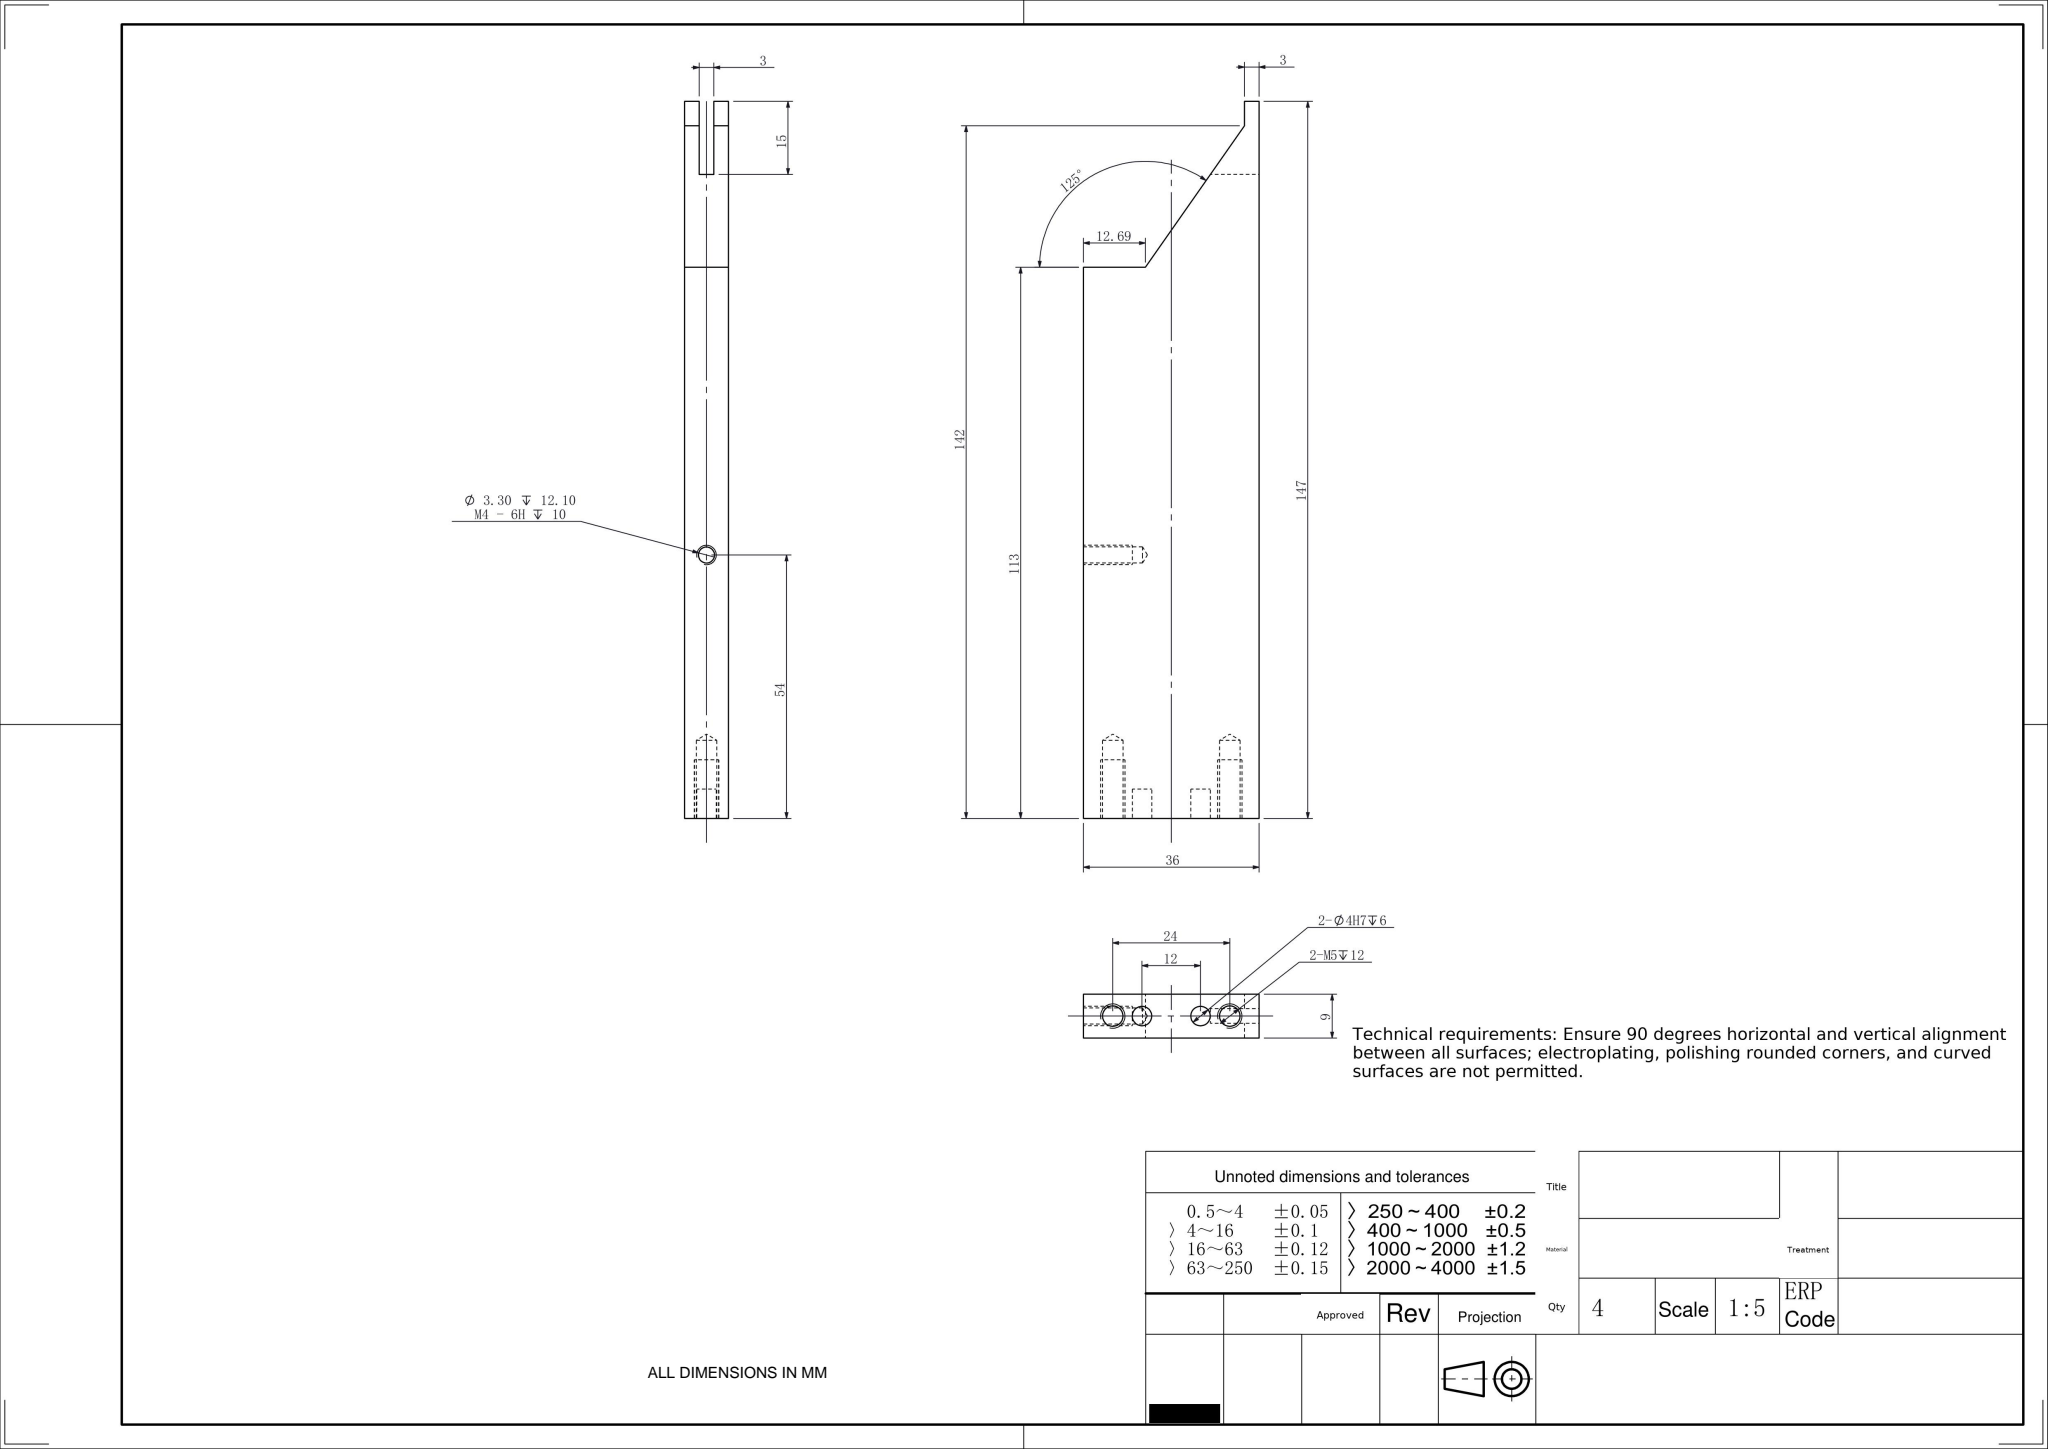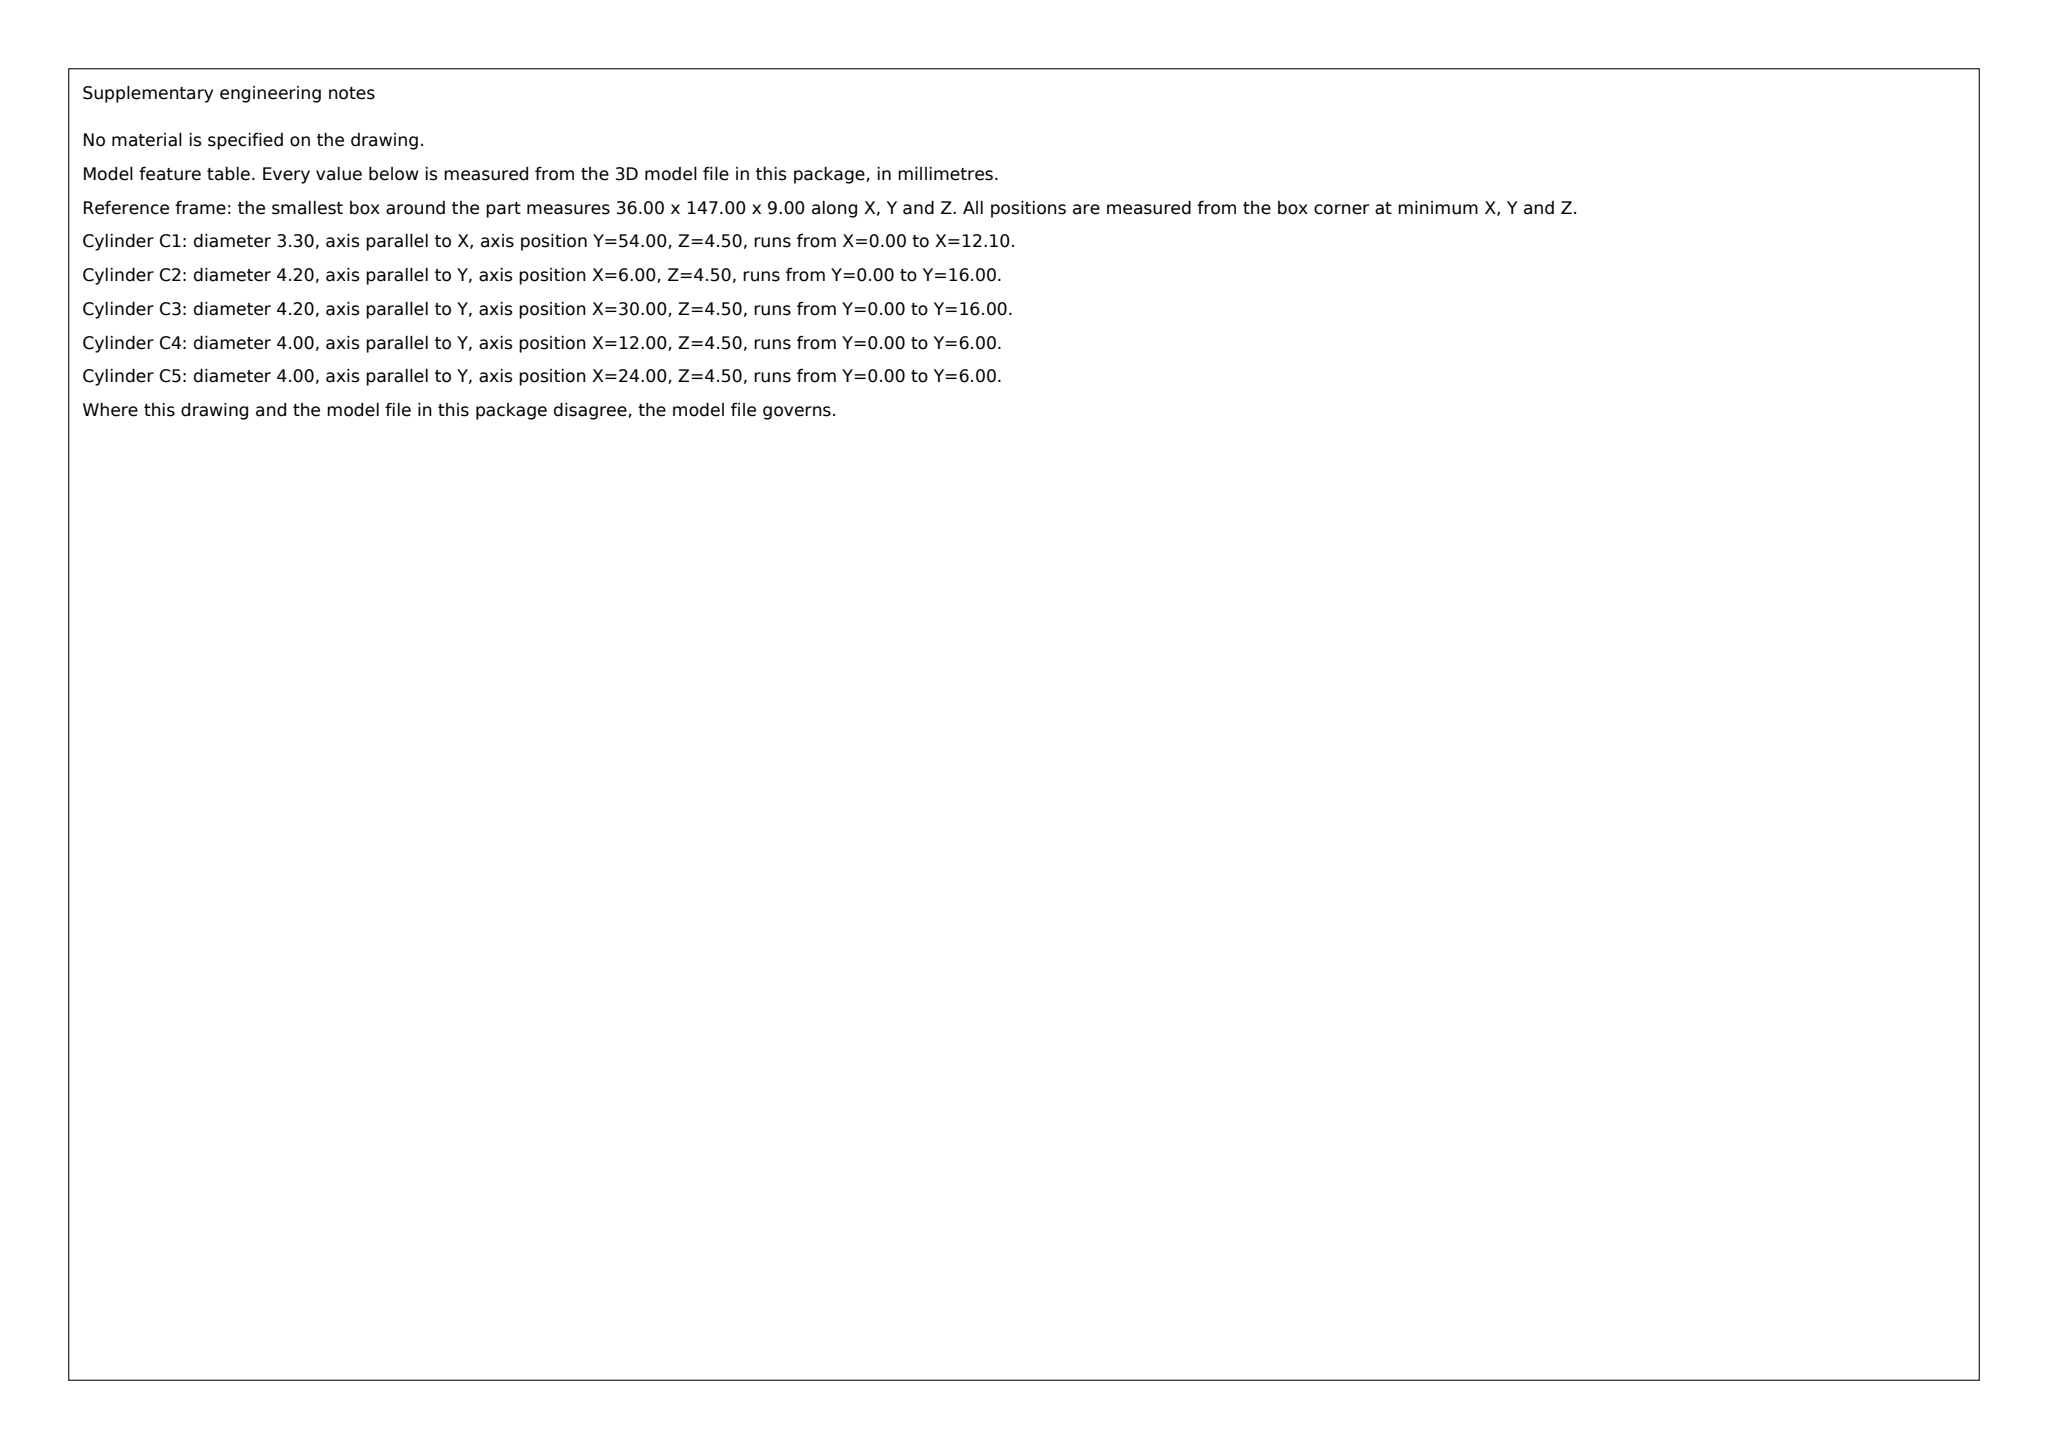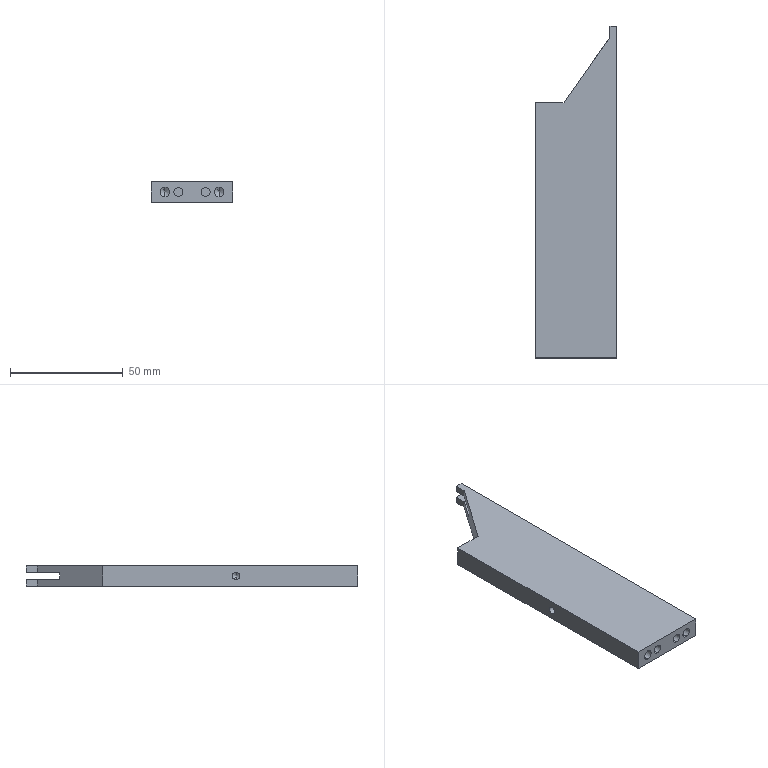Part | SolidWorks | mm | 1 solid | 32 faces | box 36 x 147 x 9 mm | volume 39228 mm3 | plane 16 | cylinder 10 | cone 6 | commonest cylinder face diameters 4 x4 4.2 x4 3.3 x2
build123d program:
from build123d import *

# Parameters (mm, degrees)
SKETCH1_W             = 36
SKETCH1_H             = 147
BOSS_EXTRUDE1_DEPTH   = 9
M5_TAPPED_HOLE1_D     = 4.2
M5_TAPPED_HOLE1_DEPTH = 16
M5_TAPPED_HOLE1_TIP   = 1.262
SKETCH3_R             = 2
CUT_EXTRUDE1_DEPTH    = 6
M4_TAPPED_HOLE1_D     = 3.3
M4_TAPPED_HOLE1_DEPTH = 12.1
M4_TAPPED_HOLE1_TIP   = 0.9914
CUT_EXTRUDE2_DEPTH    = 149.371
SKETCH8_W             = 3
SKETCH8_H             = 15
CUT_EXTRUDE3_DEPTH    = 152.611


with BuildPart() as part:
    # Sketch1 → Boss-Extrude1 (new body)
    with BuildSketch(Plane.XY):
        with Locations((0, 73.5)):
            Rectangle(SKETCH1_W, SKETCH1_H)
    extrude(amount=BOSS_EXTRUDE1_DEPTH)

    # M5 Tapped Hole1
    with Locations(Plane(origin=(-12, 0, 4.5), x_dir=(0, 0, -1), z_dir=(0, -1, 0))):
        with Locations((0, 0), (0, 24)):
            Hole(M5_TAPPED_HOLE1_D / 2, depth=M5_TAPPED_HOLE1_DEPTH)
            with Locations((0, 0, -(M5_TAPPED_HOLE1_DEPTH + M5_TAPPED_HOLE1_TIP / 2))):  # 118° drill point
                Cone(0, M5_TAPPED_HOLE1_D / 2, M5_TAPPED_HOLE1_TIP, mode=Mode.SUBTRACT)

    # Sketch3 → Cut-Extrude1 (cut)
    with BuildSketch(Plane.XZ):
        with Locations(Location((-6, 4.5, 0), (0, 0, 270))):
            Circle(SKETCH3_R)
        with Locations(Location((6, 4.5, 0), (0, 0, 270))):
            Circle(SKETCH3_R)
    extrude(amount=-CUT_EXTRUDE1_DEPTH, mode=Mode.SUBTRACT)

    # M4 Tapped Hole1
    with Locations(Plane(origin=(-18, 54, 4.5), x_dir=(0, 0, -1), z_dir=(-1, 0, 0))):
        with Locations((0, 0)):
            Hole(M4_TAPPED_HOLE1_D / 2, depth=M4_TAPPED_HOLE1_DEPTH)
            with Locations((0, 0, -(M4_TAPPED_HOLE1_DEPTH + M4_TAPPED_HOLE1_TIP / 2))):  # 118° drill point
                Cone(0, M4_TAPPED_HOLE1_D / 2, M4_TAPPED_HOLE1_TIP, mode=Mode.SUBTRACT)

    # Sketch6 → Cut-Extrude2 (cut, through all)
    with BuildSketch(Plane.XY.offset(9)):
        Polygon((15, 147), (-44.648, 147), (-44.648, 113), (-5.306, 113), (15, 142), align=None)
    extrude(amount=-CUT_EXTRUDE2_DEPTH, mode=Mode.SUBTRACT)

    # Sketch8 → Cut-Extrude3 (cut, through all)
    with BuildSketch(Plane(origin=(18, 0, 0), x_dir=(0, 0, -1), z_dir=(1, 0, 0))):
        with Locations((-4.5, 139.5)):
            Rectangle(SKETCH8_W, SKETCH8_H)
    extrude(amount=-CUT_EXTRUDE3_DEPTH, mode=Mode.SUBTRACT)


solid = part.part
STEP:
#1=CARTESIAN_POINT('',(-5.9,54.,2.85));
#2=VERTEX_POINT('',#1);
#3=CARTESIAN_POINT('',(-5.9,54.,6.15));
#4=VERTEX_POINT('',#3);
#5=CARTESIAN_POINT('',(-5.9,54.,4.5));
#6=DIRECTION('',(-1.,0.,0.));
#7=DIRECTION('',(0.,0.,1.));
#8=AXIS2_PLACEMENT_3D('',#5,#6,#7);
#9=CIRCLE('',#8,1.65);
#10=EDGE_CURVE('',#2,#4,#9,.T.);
#11=ORIENTED_EDGE('',*,*,#10,.F.);
#12=CARTESIAN_POINT('',(-18.,54.,2.85));
#13=VERTEX_POINT('',#12);
#14=CARTESIAN_POINT('',(-18.,54.,2.85));
#15=DIRECTION('',(-1.,0.,0.));
#16=VECTOR('',#15,1000.);
#17=LINE('',#14,#16);
#18=EDGE_CURVE('',#2,#13,#17,.T.);
#19=ORIENTED_EDGE('',*,*,#18,.T.);
#20=CARTESIAN_POINT('',(-18.,54.,6.15));
#21=VERTEX_POINT('',#20);
#22=CARTESIAN_POINT('',(-18.,54.,4.5));
#23=DIRECTION('',(-1.,0.,0.));
#24=DIRECTION('',(0.,0.,1.));
#25=AXIS2_PLACEMENT_3D('',#22,#23,#24);
#26=CIRCLE('',#25,1.65);
#27=EDGE_CURVE('',#13,#21,#26,.T.);
#28=ORIENTED_EDGE('',*,*,#27,.T.);
#29=CARTESIAN_POINT('',(-18.,54.,6.15));
#30=DIRECTION('',(-1.,0.,0.));
#31=VECTOR('',#30,1000.);
#32=LINE('',#29,#31);
#33=EDGE_CURVE('',#4,#21,#32,.T.);
#34=ORIENTED_EDGE('',*,*,#33,.F.);
#35=EDGE_LOOP('',(#11,#19,#28,#34));
#36=FACE_OUTER_BOUND('',#35,.T.);
#37=CARTESIAN_POINT('',(-18.,54.,4.5));
#38=DIRECTION('',(-1.,0.,0.));
#39=DIRECTION('',(0.,0.,1.));
#40=AXIS2_PLACEMENT_3D('',#37,#38,#39);
#41=CYLINDRICAL_SURFACE('',#40,1.65);
#42=ADVANCED_FACE('',(#36),#41,.F.);
#43=CARTESIAN_POINT('',(-4.909,54.,4.5));
#44=VERTEX_POINT('',#43);
#45=CARTESIAN_POINT('',(-5.9,54.,6.15));
#46=DIRECTION('',(-0.515,0.,0.8572));
#47=VECTOR('',#46,1000.);
#48=LINE('',#45,#47);
#49=EDGE_CURVE('',#44,#4,#48,.T.);
#50=ORIENTED_EDGE('',*,*,#49,.F.);
#51=CARTESIAN_POINT('',(-5.9,54.,2.85));
#52=DIRECTION('',(-0.515,0.,-0.8572));
#53=VECTOR('',#52,1000.);
#54=LINE('',#51,#53);
#55=EDGE_CURVE('',#44,#2,#54,.T.);
#56=ORIENTED_EDGE('',*,*,#55,.T.);
#57=ORIENTED_EDGE('',*,*,#10,.T.);
#58=EDGE_LOOP('',(#50,#56,#57));
#59=FACE_OUTER_BOUND('',#58,.T.);
#60=CARTESIAN_POINT('',(-5.9,54.,4.5));
#61=DIRECTION('',(-1.,0.,0.));
#62=DIRECTION('',(0.,0.,1.));
#63=AXIS2_PLACEMENT_3D('',#60,#61,#62);
#64=CONICAL_SURFACE('',#63,1.65,1.03);
#65=ADVANCED_FACE('',(#59),#64,.F.);
#66=CARTESIAN_POINT('',(6.,6.,6.5));
#67=VERTEX_POINT('',#66);
#68=CARTESIAN_POINT('',(6.,6.,2.5));
#69=VERTEX_POINT('',#68);
#70=CARTESIAN_POINT('',(6.,6.,4.5));
#71=DIRECTION('',(0.,-1.,0.));
#72=DIRECTION('',(0.,0.,-1.));
#73=AXIS2_PLACEMENT_3D('',#70,#71,#72);
#74=CIRCLE('',#73,2.);
#75=EDGE_CURVE('',#67,#69,#74,.T.);
#76=ORIENTED_EDGE('',*,*,#75,.F.);
#77=CARTESIAN_POINT('',(6.,0.,6.5));
#78=VERTEX_POINT('',#77);
#79=CARTESIAN_POINT('',(6.,6.,6.5));
#80=DIRECTION('',(0.,-1.,0.));
#81=VECTOR('',#80,1000.);
#82=LINE('',#79,#81);
#83=EDGE_CURVE('',#67,#78,#82,.T.);
#84=ORIENTED_EDGE('',*,*,#83,.T.);
#85=CARTESIAN_POINT('',(6.,0.,2.5));
#86=VERTEX_POINT('',#85);
#87=CARTESIAN_POINT('',(6.,0.,4.5));
#88=DIRECTION('',(0.,-1.,0.));
#89=DIRECTION('',(0.,0.,-1.));
#90=AXIS2_PLACEMENT_3D('',#87,#88,#89);
#91=CIRCLE('',#90,2.);
#92=EDGE_CURVE('',#78,#86,#91,.T.);
#93=ORIENTED_EDGE('',*,*,#92,.T.);
#94=CARTESIAN_POINT('',(6.,6.,2.5));
#95=DIRECTION('',(0.,-1.,0.));
#96=VECTOR('',#95,1000.);
#97=LINE('',#94,#96);
#98=EDGE_CURVE('',#69,#86,#97,.T.);
#99=ORIENTED_EDGE('',*,*,#98,.F.);
#100=EDGE_LOOP('',(#76,#84,#93,#99));
#101=FACE_OUTER_BOUND('',#100,.T.);
#102=CARTESIAN_POINT('',(6.,6.,4.5));
#103=DIRECTION('',(0.,-1.,0.));
#104=DIRECTION('',(0.,0.,-1.));
#105=AXIS2_PLACEMENT_3D('',#102,#103,#104);
#106=CYLINDRICAL_SURFACE('',#105,2.);
#107=ADVANCED_FACE('',(#101),#106,.F.);
#108=CARTESIAN_POINT('',(-6.,6.,6.5));
#109=VERTEX_POINT('',#108);
#110=CARTESIAN_POINT('',(-6.,6.,2.5));
#111=VERTEX_POINT('',#110);
#112=CARTESIAN_POINT('',(-6.,6.,4.5));
#113=DIRECTION('',(0.,-1.,0.));
#114=DIRECTION('',(0.,0.,-1.));
#115=AXIS2_PLACEMENT_3D('',#112,#113,#114);
#116=CIRCLE('',#115,2.);
#117=EDGE_CURVE('',#109,#111,#116,.T.);
#118=ORIENTED_EDGE('',*,*,#117,.F.);
#119=CARTESIAN_POINT('',(-6.,0.,6.5));
#120=VERTEX_POINT('',#119);
#121=CARTESIAN_POINT('',(-6.,6.,6.5));
#122=DIRECTION('',(0.,-1.,0.));
#123=VECTOR('',#122,1000.);
#124=LINE('',#121,#123);
#125=EDGE_CURVE('',#109,#120,#124,.T.);
#126=ORIENTED_EDGE('',*,*,#125,.T.);
#127=CARTESIAN_POINT('',(-6.,0.,2.5));
#128=VERTEX_POINT('',#127);
#129=CARTESIAN_POINT('',(-6.,0.,4.5));
#130=DIRECTION('',(0.,-1.,0.));
#131=DIRECTION('',(0.,0.,-1.));
#132=AXIS2_PLACEMENT_3D('',#129,#130,#131);
#133=CIRCLE('',#132,2.);
#134=EDGE_CURVE('',#120,#128,#133,.T.);
#135=ORIENTED_EDGE('',*,*,#134,.T.);
#136=CARTESIAN_POINT('',(-6.,6.,2.5));
#137=DIRECTION('',(0.,-1.,0.));
#138=VECTOR('',#137,1000.);
#139=LINE('',#136,#138);
#140=EDGE_CURVE('',#111,#128,#139,.T.);
#141=ORIENTED_EDGE('',*,*,#140,.F.);
#142=EDGE_LOOP('',(#118,#126,#135,#141));
#143=FACE_OUTER_BOUND('',#142,.T.);
#144=CARTESIAN_POINT('',(-6.,6.,4.5));
#145=DIRECTION('',(0.,-1.,0.));
#146=DIRECTION('',(0.,0.,-1.));
#147=AXIS2_PLACEMENT_3D('',#144,#145,#146);
#148=CYLINDRICAL_SURFACE('',#147,2.);
#149=ADVANCED_FACE('',(#143),#148,.F.);
#150=CARTESIAN_POINT('',(-12.,16.,6.6));
#151=VERTEX_POINT('',#150);
#152=CARTESIAN_POINT('',(-12.,16.,2.4));
#153=VERTEX_POINT('',#152);
#154=CARTESIAN_POINT('',(-12.,16.,4.5));
#155=DIRECTION('',(0.,-1.,0.));
#156=DIRECTION('',(0.,0.,-1.));
#157=AXIS2_PLACEMENT_3D('',#154,#155,#156);
#158=CIRCLE('',#157,2.1);
#159=EDGE_CURVE('',#151,#153,#158,.T.);
#160=ORIENTED_EDGE('',*,*,#159,.F.);
#161=CARTESIAN_POINT('',(-12.,-0.,6.6));
#162=VERTEX_POINT('',#161);
#163=CARTESIAN_POINT('',(-12.,0.,6.6));
#164=DIRECTION('',(0.,-1.,0.));
#165=VECTOR('',#164,1000.);
#166=LINE('',#163,#165);
#167=EDGE_CURVE('',#151,#162,#166,.T.);
#168=ORIENTED_EDGE('',*,*,#167,.T.);
#169=CARTESIAN_POINT('',(-12.,-0.,2.4));
#170=VERTEX_POINT('',#169);
#171=CARTESIAN_POINT('',(-12.,-0.,4.5));
#172=DIRECTION('',(0.,-1.,0.));
#173=DIRECTION('',(0.,0.,-1.));
#174=AXIS2_PLACEMENT_3D('',#171,#172,#173);
#175=CIRCLE('',#174,2.1);
#176=EDGE_CURVE('',#162,#170,#175,.T.);
#177=ORIENTED_EDGE('',*,*,#176,.T.);
#178=CARTESIAN_POINT('',(-12.,0.,2.4));
#179=DIRECTION('',(0.,-1.,0.));
#180=VECTOR('',#179,1000.);
#181=LINE('',#178,#180);
#182=EDGE_CURVE('',#153,#170,#181,.T.);
#183=ORIENTED_EDGE('',*,*,#182,.F.);
#184=EDGE_LOOP('',(#160,#168,#177,#183));
#185=FACE_OUTER_BOUND('',#184,.T.);
#186=CARTESIAN_POINT('',(-12.,0.,4.5));
#187=DIRECTION('',(0.,-1.,0.));
#188=DIRECTION('',(0.,0.,-1.));
#189=AXIS2_PLACEMENT_3D('',#186,#187,#188);
#190=CYLINDRICAL_SURFACE('',#189,2.1);
#191=ADVANCED_FACE('',(#185),#190,.F.);
#192=CARTESIAN_POINT('',(-12.,17.262,4.5));
#193=VERTEX_POINT('',#192);
#194=CARTESIAN_POINT('',(-12.,16.,2.4));
#195=DIRECTION('',(0.,-0.515,-0.8572));
#196=VECTOR('',#195,1000.);
#197=LINE('',#194,#196);
#198=EDGE_CURVE('',#193,#153,#197,.T.);
#199=ORIENTED_EDGE('',*,*,#198,.F.);
#200=CARTESIAN_POINT('',(-12.,16.,6.6));
#201=DIRECTION('',(0.,-0.515,0.8572));
#202=VECTOR('',#201,1000.);
#203=LINE('',#200,#202);
#204=EDGE_CURVE('',#193,#151,#203,.T.);
#205=ORIENTED_EDGE('',*,*,#204,.T.);
#206=ORIENTED_EDGE('',*,*,#159,.T.);
#207=EDGE_LOOP('',(#199,#205,#206));
#208=FACE_OUTER_BOUND('',#207,.T.);
#209=CARTESIAN_POINT('',(-12.,16.,4.5));
#210=DIRECTION('',(0.,-1.,0.));
#211=DIRECTION('',(0.,0.,-1.));
#212=AXIS2_PLACEMENT_3D('',#209,#210,#211);
#213=CONICAL_SURFACE('',#212,2.1,1.03);
#214=ADVANCED_FACE('',(#208),#213,.F.);
#215=CARTESIAN_POINT('',(12.,16.,6.6));
#216=VERTEX_POINT('',#215);
#217=CARTESIAN_POINT('',(12.,16.,2.4));
#218=VERTEX_POINT('',#217);
#219=CARTESIAN_POINT('',(12.,16.,4.5));
#220=DIRECTION('',(0.,-1.,0.));
#221=DIRECTION('',(0.,0.,-1.));
#222=AXIS2_PLACEMENT_3D('',#219,#220,#221);
#223=CIRCLE('',#222,2.1);
#224=EDGE_CURVE('',#216,#218,#223,.T.);
#225=ORIENTED_EDGE('',*,*,#224,.F.);
#226=CARTESIAN_POINT('',(12.,-0.,6.6));
#227=VERTEX_POINT('',#226);
#228=CARTESIAN_POINT('',(12.,0.,6.6));
#229=DIRECTION('',(0.,-1.,0.));
#230=VECTOR('',#229,1000.);
#231=LINE('',#228,#230);
#232=EDGE_CURVE('',#216,#227,#231,.T.);
#233=ORIENTED_EDGE('',*,*,#232,.T.);
#234=CARTESIAN_POINT('',(12.,-0.,2.4));
#235=VERTEX_POINT('',#234);
#236=CARTESIAN_POINT('',(12.,-0.,4.5));
#237=DIRECTION('',(0.,-1.,0.));
#238=DIRECTION('',(0.,0.,-1.));
#239=AXIS2_PLACEMENT_3D('',#236,#237,#238);
#240=CIRCLE('',#239,2.1);
#241=EDGE_CURVE('',#227,#235,#240,.T.);
#242=ORIENTED_EDGE('',*,*,#241,.T.);
#243=CARTESIAN_POINT('',(12.,0.,2.4));
#244=DIRECTION('',(0.,-1.,0.));
#245=VECTOR('',#244,1000.);
#246=LINE('',#243,#245);
#247=EDGE_CURVE('',#218,#235,#246,.T.);
#248=ORIENTED_EDGE('',*,*,#247,.F.);
#249=EDGE_LOOP('',(#225,#233,#242,#248));
#250=FACE_OUTER_BOUND('',#249,.T.);
#251=CARTESIAN_POINT('',(12.,0.,4.5));
#252=DIRECTION('',(0.,-1.,0.));
#253=DIRECTION('',(0.,0.,-1.));
#254=AXIS2_PLACEMENT_3D('',#251,#252,#253);
#255=CYLINDRICAL_SURFACE('',#254,2.1);
#256=ADVANCED_FACE('',(#250),#255,.F.);
#257=CARTESIAN_POINT('',(12.,17.262,4.5));
#258=VERTEX_POINT('',#257);
#259=CARTESIAN_POINT('',(12.,16.,2.4));
#260=DIRECTION('',(0.,-0.515,-0.8572));
#261=VECTOR('',#260,1000.);
#262=LINE('',#259,#261);
#263=EDGE_CURVE('',#258,#218,#262,.T.);
#264=ORIENTED_EDGE('',*,*,#263,.F.);
#265=CARTESIAN_POINT('',(12.,16.,6.6));
#266=DIRECTION('',(0.,-0.515,0.8572));
#267=VECTOR('',#266,1000.);
#268=LINE('',#265,#267);
#269=EDGE_CURVE('',#258,#216,#268,.T.);
#270=ORIENTED_EDGE('',*,*,#269,.T.);
#271=ORIENTED_EDGE('',*,*,#224,.T.);
#272=EDGE_LOOP('',(#264,#270,#271));
#273=FACE_OUTER_BOUND('',#272,.T.);
#274=CARTESIAN_POINT('',(12.,16.,4.5));
#275=DIRECTION('',(0.,-1.,0.));
#276=DIRECTION('',(0.,0.,-1.));
#277=AXIS2_PLACEMENT_3D('',#274,#275,#276);
#278=CONICAL_SURFACE('',#277,2.1,1.03);
#279=ADVANCED_FACE('',(#273),#278,.F.);
#280=CARTESIAN_POINT('',(18.,147.,9.));
#281=VERTEX_POINT('',#280);
#282=CARTESIAN_POINT('',(18.,147.,6.));
#283=VERTEX_POINT('',#282);
#284=CARTESIAN_POINT('',(18.,147.,9.));
#285=DIRECTION('',(0.,0.,-1.));
#286=VECTOR('',#285,1000.);
#287=LINE('',#284,#286);
#288=EDGE_CURVE('',#281,#283,#287,.T.);
#289=ORIENTED_EDGE('',*,*,#288,.T.);
#290=CARTESIAN_POINT('',(15.,147.,6.));
#291=VERTEX_POINT('',#290);
#292=CARTESIAN_POINT('',(-18.,147.,6.));
#293=DIRECTION('',(1.,0.,0.));
#294=VECTOR('',#293,1000.);
#295=LINE('',#292,#294);
#296=EDGE_CURVE('',#291,#283,#295,.T.);
#297=ORIENTED_EDGE('',*,*,#296,.F.);
#298=CARTESIAN_POINT('',(15.,147.,9.));
#299=VERTEX_POINT('',#298);
#300=CARTESIAN_POINT('',(15.,147.,0.));
#301=DIRECTION('',(0.,0.,1.));
#302=VECTOR('',#301,1000.);
#303=LINE('',#300,#302);
#304=EDGE_CURVE('',#291,#299,#303,.T.);
#305=ORIENTED_EDGE('',*,*,#304,.T.);
#306=CARTESIAN_POINT('',(-18.,147.,9.));
#307=DIRECTION('',(-1.,0.,0.));
#308=VECTOR('',#307,1000.);
#309=LINE('',#306,#308);
#310=EDGE_CURVE('',#281,#299,#309,.T.);
#311=ORIENTED_EDGE('',*,*,#310,.F.);
#312=EDGE_LOOP('',(#289,#297,#305,#311));
#313=FACE_OUTER_BOUND('',#312,.T.);
#314=CARTESIAN_POINT('',(-18.,147.,9.));
#315=DIRECTION('',(-0.,-1.,0.));
#316=DIRECTION('',(1.,-0.,0.));
#317=AXIS2_PLACEMENT_3D('',#314,#315,#316);
#318=PLANE('',#317);
#319=ADVANCED_FACE('',(#313),#318,.F.);
#320=ORIENTED_EDGE('',*,*,#304,.F.);
#321=CARTESIAN_POINT('',(15.,142.,6.));
#322=VERTEX_POINT('',#321);
#323=CARTESIAN_POINT('',(15.,147.,6.));
#324=DIRECTION('',(0.,-1.,0.));
#325=VECTOR('',#324,1000.);
#326=LINE('',#323,#325);
#327=EDGE_CURVE('',#291,#322,#326,.T.);
#328=ORIENTED_EDGE('',*,*,#327,.T.);
#329=CARTESIAN_POINT('',(15.,142.,9.));
#330=VERTEX_POINT('',#329);
#331=CARTESIAN_POINT('',(15.,142.,0.));
#332=DIRECTION('',(0.,0.,1.));
#333=VECTOR('',#332,1000.);
#334=LINE('',#331,#333);
#335=EDGE_CURVE('',#322,#330,#334,.T.);
#336=ORIENTED_EDGE('',*,*,#335,.T.);
#337=CARTESIAN_POINT('',(15.,147.,9.));
#338=DIRECTION('',(0.,1.,0.));
#339=VECTOR('',#338,1000.);
#340=LINE('',#337,#339);
#341=EDGE_CURVE('',#330,#299,#340,.T.);
#342=ORIENTED_EDGE('',*,*,#341,.T.);
#343=EDGE_LOOP('',(#320,#328,#336,#342));
#344=FACE_OUTER_BOUND('',#343,.T.);
#345=CARTESIAN_POINT('',(15.,147.,0.));
#346=DIRECTION('',(1.,0.,0.));
#347=DIRECTION('',(0.,0.,-1.));
#348=AXIS2_PLACEMENT_3D('',#345,#346,#347);
#349=PLANE('',#348);
#350=ADVANCED_FACE('',(#344),#349,.F.);
#351=CARTESIAN_POINT('',(-18.,54.,4.5));
#352=DIRECTION('',(-1.,0.,0.));
#353=DIRECTION('',(0.,0.,1.));
#354=AXIS2_PLACEMENT_3D('',#351,#352,#353);
#355=CIRCLE('',#354,1.65);
#356=EDGE_CURVE('',#21,#13,#355,.T.);
#357=ORIENTED_EDGE('',*,*,#356,.F.);
#358=ORIENTED_EDGE('',*,*,#27,.F.);
#359=EDGE_LOOP('',(#357,#358));
#360=FACE_BOUND('',#359,.T.);
#361=CARTESIAN_POINT('',(-18.,113.,9.));
#362=VERTEX_POINT('',#361);
#363=CARTESIAN_POINT('',(-18.,0.,9.));
#364=VERTEX_POINT('',#363);
#365=CARTESIAN_POINT('',(-18.,0.,9.));
#366=DIRECTION('',(0.,-1.,0.));
#367=VECTOR('',#366,1000.);
#368=LINE('',#365,#367);
#369=EDGE_CURVE('',#362,#364,#368,.T.);
#370=ORIENTED_EDGE('',*,*,#369,.F.);
#371=CARTESIAN_POINT('',(-18.,113.,0.));
#372=VERTEX_POINT('',#371);
#373=CARTESIAN_POINT('',(-18.,113.,9.));
#374=DIRECTION('',(0.,0.,-1.));
#375=VECTOR('',#374,1000.);
#376=LINE('',#373,#375);
#377=EDGE_CURVE('',#362,#372,#376,.T.);
#378=ORIENTED_EDGE('',*,*,#377,.T.);
#379=CARTESIAN_POINT('',(-18.,0.,0.));
#380=VERTEX_POINT('',#379);
#381=CARTESIAN_POINT('',(-18.,0.,0.));
#382=DIRECTION('',(0.,-1.,0.));
#383=VECTOR('',#382,1000.);
#384=LINE('',#381,#383);
#385=EDGE_CURVE('',#372,#380,#384,.T.);
#386=ORIENTED_EDGE('',*,*,#385,.T.);
#387=CARTESIAN_POINT('',(-18.,0.,9.));
#388=DIRECTION('',(0.,0.,-1.));
#389=VECTOR('',#388,1000.);
#390=LINE('',#387,#389);
#391=EDGE_CURVE('',#364,#380,#390,.T.);
#392=ORIENTED_EDGE('',*,*,#391,.F.);
#393=EDGE_LOOP('',(#370,#378,#386,#392));
#394=FACE_OUTER_BOUND('',#393,.T.);
#395=CARTESIAN_POINT('',(-18.,0.,9.));
#396=DIRECTION('',(1.,0.,0.));
#397=DIRECTION('',(0.,0.,-1.));
#398=AXIS2_PLACEMENT_3D('',#395,#396,#397);
#399=PLANE('',#398);
#400=ADVANCED_FACE('',(#360,#394),#399,.F.);
#401=CARTESIAN_POINT('',(6.,0.,4.5));
#402=DIRECTION('',(0.,-1.,0.));
#403=DIRECTION('',(0.,0.,-1.));
#404=AXIS2_PLACEMENT_3D('',#401,#402,#403);
#405=CIRCLE('',#404,2.);
#406=EDGE_CURVE('',#86,#78,#405,.T.);
#407=ORIENTED_EDGE('',*,*,#406,.F.);
#408=ORIENTED_EDGE('',*,*,#92,.F.);
#409=EDGE_LOOP('',(#407,#408));
#410=FACE_BOUND('',#409,.T.);
#411=CARTESIAN_POINT('',(-6.,0.,4.5));
#412=DIRECTION('',(0.,-1.,0.));
#413=DIRECTION('',(0.,0.,-1.));
#414=AXIS2_PLACEMENT_3D('',#411,#412,#413);
#415=CIRCLE('',#414,2.);
#416=EDGE_CURVE('',#128,#120,#415,.T.);
#417=ORIENTED_EDGE('',*,*,#416,.F.);
#418=ORIENTED_EDGE('',*,*,#134,.F.);
#419=EDGE_LOOP('',(#417,#418));
#420=FACE_BOUND('',#419,.T.);
#421=CARTESIAN_POINT('',(-12.,-0.,4.5));
#422=DIRECTION('',(0.,-1.,0.));
#423=DIRECTION('',(0.,0.,-1.));
#424=AXIS2_PLACEMENT_3D('',#421,#422,#423);
#425=CIRCLE('',#424,2.1);
#426=EDGE_CURVE('',#170,#162,#425,.T.);
#427=ORIENTED_EDGE('',*,*,#426,.F.);
#428=ORIENTED_EDGE('',*,*,#176,.F.);
#429=EDGE_LOOP('',(#427,#428));
#430=FACE_BOUND('',#429,.T.);
#431=CARTESIAN_POINT('',(12.,-0.,4.5));
#432=DIRECTION('',(0.,-1.,0.));
#433=DIRECTION('',(0.,0.,-1.));
#434=AXIS2_PLACEMENT_3D('',#431,#432,#433);
#435=CIRCLE('',#434,2.1);
#436=EDGE_CURVE('',#235,#227,#435,.T.);
#437=ORIENTED_EDGE('',*,*,#436,.F.);
#438=ORIENTED_EDGE('',*,*,#241,.F.);
#439=EDGE_LOOP('',(#437,#438));
#440=FACE_BOUND('',#439,.T.);
#441=CARTESIAN_POINT('',(18.,0.,0.));
#442=VERTEX_POINT('',#441);
#443=CARTESIAN_POINT('',(-18.,0.,0.));
#444=DIRECTION('',(1.,0.,0.));
#445=VECTOR('',#444,1000.);
#446=LINE('',#443,#445);
#447=EDGE_CURVE('',#380,#442,#446,.T.);
#448=ORIENTED_EDGE('',*,*,#447,.T.);
#449=CARTESIAN_POINT('',(18.,0.,9.));
#450=VERTEX_POINT('',#449);
#451=CARTESIAN_POINT('',(18.,0.,9.));
#452=DIRECTION('',(0.,0.,-1.));
#453=VECTOR('',#452,1000.);
#454=LINE('',#451,#453);
#455=EDGE_CURVE('',#450,#442,#454,.T.);
#456=ORIENTED_EDGE('',*,*,#455,.F.);
#457=CARTESIAN_POINT('',(-18.,0.,9.));
#458=DIRECTION('',(1.,0.,0.));
#459=VECTOR('',#458,1000.);
#460=LINE('',#457,#459);
#461=EDGE_CURVE('',#364,#450,#460,.T.);
#462=ORIENTED_EDGE('',*,*,#461,.F.);
#463=ORIENTED_EDGE('',*,*,#391,.T.);
#464=EDGE_LOOP('',(#448,#456,#462,#463));
#465=FACE_OUTER_BOUND('',#464,.T.);
#466=CARTESIAN_POINT('',(-18.,0.,9.));
#467=DIRECTION('',(0.,1.,0.));
#468=DIRECTION('',(0.,0.,1.));
#469=AXIS2_PLACEMENT_3D('',#466,#467,#468);
#470=PLANE('',#469);
#471=ADVANCED_FACE('',(#410,#420,#430,#440,#465),#470,.F.);
#472=CARTESIAN_POINT('',(18.,132.,6.));
#473=VERTEX_POINT('',#472);
#474=CARTESIAN_POINT('',(18.,132.,3.));
#475=VERTEX_POINT('',#474);
#476=CARTESIAN_POINT('',(18.,132.,6.));
#477=DIRECTION('',(0.,0.,-1.));
#478=VECTOR('',#477,1000.);
#479=LINE('',#476,#478);
#480=EDGE_CURVE('',#473,#475,#479,.T.);
#481=ORIENTED_EDGE('',*,*,#480,.F.);
#482=CARTESIAN_POINT('',(18.,147.,6.));
#483=DIRECTION('',(0.,-1.,0.));
#484=VECTOR('',#483,1000.);
#485=LINE('',#482,#484);
#486=EDGE_CURVE('',#283,#473,#485,.T.);
#487=ORIENTED_EDGE('',*,*,#486,.F.);
#488=ORIENTED_EDGE('',*,*,#288,.F.);
#489=CARTESIAN_POINT('',(18.,0.,9.));
#490=DIRECTION('',(0.,1.,0.));
#491=VECTOR('',#490,1000.);
#492=LINE('',#489,#491);
#493=EDGE_CURVE('',#450,#281,#492,.T.);
#494=ORIENTED_EDGE('',*,*,#493,.F.);
#495=ORIENTED_EDGE('',*,*,#455,.T.);
#496=CARTESIAN_POINT('',(18.,147.,0.));
#497=VERTEX_POINT('',#496);
#498=CARTESIAN_POINT('',(18.,0.,0.));
#499=DIRECTION('',(0.,1.,0.));
#500=VECTOR('',#499,1000.);
#501=LINE('',#498,#500);
#502=EDGE_CURVE('',#442,#497,#501,.T.);
#503=ORIENTED_EDGE('',*,*,#502,.T.);
#504=CARTESIAN_POINT('',(18.,147.,3.));
#505=VERTEX_POINT('',#504);
#506=CARTESIAN_POINT('',(18.,147.,9.));
#507=DIRECTION('',(0.,0.,-1.));
#508=VECTOR('',#507,1000.);
#509=LINE('',#506,#508);
#510=EDGE_CURVE('',#505,#497,#509,.T.);
#511=ORIENTED_EDGE('',*,*,#510,.F.);
#512=CARTESIAN_POINT('',(18.,147.,3.));
#513=DIRECTION('',(0.,1.,0.));
#514=VECTOR('',#513,1000.);
#515=LINE('',#512,#514);
#516=EDGE_CURVE('',#475,#505,#515,.T.);
#517=ORIENTED_EDGE('',*,*,#516,.F.);
#518=EDGE_LOOP('',(#481,#487,#488,#494,#495,#503,#511,#517));
#519=FACE_OUTER_BOUND('',#518,.T.);
#520=CARTESIAN_POINT('',(18.,0.,9.));
#521=DIRECTION('',(-1.,0.,0.));
#522=DIRECTION('',(0.,0.,1.));
#523=AXIS2_PLACEMENT_3D('',#520,#521,#522);
#524=PLANE('',#523);
#525=ADVANCED_FACE('',(#519),#524,.F.);
#526=CARTESIAN_POINT('',(15.,147.,0.));
#527=VERTEX_POINT('',#526);
#528=CARTESIAN_POINT('',(15.,147.,3.));
#529=VERTEX_POINT('',#528);
#530=CARTESIAN_POINT('',(15.,147.,0.));
#531=DIRECTION('',(0.,0.,1.));
#532=VECTOR('',#531,1000.);
#533=LINE('',#530,#532);
#534=EDGE_CURVE('',#527,#529,#533,.T.);
#535=ORIENTED_EDGE('',*,*,#534,.T.);
#536=CARTESIAN_POINT('',(-18.,147.,3.));
#537=DIRECTION('',(1.,0.,0.));
#538=VECTOR('',#537,1000.);
#539=LINE('',#536,#538);
#540=EDGE_CURVE('',#529,#505,#539,.T.);
#541=ORIENTED_EDGE('',*,*,#540,.T.);
#542=ORIENTED_EDGE('',*,*,#510,.T.);
#543=CARTESIAN_POINT('',(-18.,147.,0.));
#544=DIRECTION('',(-1.,0.,0.));
#545=VECTOR('',#544,1000.);
#546=LINE('',#543,#545);
#547=EDGE_CURVE('',#497,#527,#546,.T.);
#548=ORIENTED_EDGE('',*,*,#547,.T.);
#549=EDGE_LOOP('',(#535,#541,#542,#548));
#550=FACE_OUTER_BOUND('',#549,.T.);
#551=CARTESIAN_POINT('',(-18.,147.,9.));
#552=DIRECTION('',(-0.,-1.,0.));
#553=DIRECTION('',(1.,-0.,0.));
#554=AXIS2_PLACEMENT_3D('',#551,#552,#553);
#555=PLANE('',#554);
#556=ADVANCED_FACE('',(#550),#555,.F.);
#557=ORIENTED_EDGE('',*,*,#310,.T.);
#558=ORIENTED_EDGE('',*,*,#341,.F.);
#559=CARTESIAN_POINT('',(-5.306,113.,9.));
#560=VERTEX_POINT('',#559);
#561=CARTESIAN_POINT('',(15.,142.,9.));
#562=DIRECTION('',(0.5736,0.8192,0.));
#563=VECTOR('',#562,1000.);
#564=LINE('',#561,#563);
#565=EDGE_CURVE('',#560,#330,#564,.T.);
#566=ORIENTED_EDGE('',*,*,#565,.F.);
#567=CARTESIAN_POINT('',(-5.306,113.,9.));
#568=DIRECTION('',(1.,0.,0.));
#569=VECTOR('',#568,1000.);
#570=LINE('',#567,#569);
#571=EDGE_CURVE('',#362,#560,#570,.T.);
#572=ORIENTED_EDGE('',*,*,#571,.F.);
#573=ORIENTED_EDGE('',*,*,#369,.T.);
#574=ORIENTED_EDGE('',*,*,#461,.T.);
#575=ORIENTED_EDGE('',*,*,#493,.T.);
#576=EDGE_LOOP('',(#557,#558,#566,#572,#573,#574,#575));
#577=FACE_OUTER_BOUND('',#576,.T.);
#578=CARTESIAN_POINT('',(-18.,147.,9.));
#579=DIRECTION('',(0.,0.,-1.));
#580=DIRECTION('',(-1.,0.,0.));
#581=AXIS2_PLACEMENT_3D('',#578,#579,#580);
#582=PLANE('',#581);
#583=ADVANCED_FACE('',(#577),#582,.F.);
#584=CARTESIAN_POINT('',(15.,142.,0.));
#585=VERTEX_POINT('',#584);
#586=CARTESIAN_POINT('',(15.,147.,0.));
#587=DIRECTION('',(0.,1.,0.));
#588=VECTOR('',#587,1000.);
#589=LINE('',#586,#588);
#590=EDGE_CURVE('',#585,#527,#589,.T.);
#591=ORIENTED_EDGE('',*,*,#590,.T.);
#592=ORIENTED_EDGE('',*,*,#547,.F.);
#593=ORIENTED_EDGE('',*,*,#502,.F.);
#594=ORIENTED_EDGE('',*,*,#447,.F.);
#595=ORIENTED_EDGE('',*,*,#385,.F.);
#596=CARTESIAN_POINT('',(-5.306,113.,0.));
#597=VERTEX_POINT('',#596);
#598=CARTESIAN_POINT('',(-18.,113.,0.));
#599=DIRECTION('',(-1.,0.,0.));
#600=VECTOR('',#599,1000.);
#601=LINE('',#598,#600);
#602=EDGE_CURVE('',#597,#372,#601,.T.);
#603=ORIENTED_EDGE('',*,*,#602,.F.);
#604=CARTESIAN_POINT('',(15.,142.,0.));
#605=DIRECTION('',(0.5736,0.8192,0.));
#606=VECTOR('',#605,1000.);
#607=LINE('',#604,#606);
#608=EDGE_CURVE('',#597,#585,#607,.T.);
#609=ORIENTED_EDGE('',*,*,#608,.T.);
#610=EDGE_LOOP('',(#591,#592,#593,#594,#595,#603,#609));
#611=FACE_OUTER_BOUND('',#610,.T.);
#612=CARTESIAN_POINT('',(-18.,147.,0.));
#613=DIRECTION('',(0.,0.,-1.));
#614=DIRECTION('',(-1.,0.,0.));
#615=AXIS2_PLACEMENT_3D('',#612,#613,#614);
#616=PLANE('',#615);
#617=ADVANCED_FACE('',(#611),#616,.T.);
#618=ORIENTED_EDGE('',*,*,#269,.F.);
#619=ORIENTED_EDGE('',*,*,#263,.T.);
#620=CARTESIAN_POINT('',(12.,16.,4.5));
#621=DIRECTION('',(0.,-1.,0.));
#622=DIRECTION('',(0.,0.,-1.));
#623=AXIS2_PLACEMENT_3D('',#620,#621,#622);
#624=CIRCLE('',#623,2.1);
#625=EDGE_CURVE('',#218,#216,#624,.T.);
#626=ORIENTED_EDGE('',*,*,#625,.T.);
#627=EDGE_LOOP('',(#618,#619,#626));
#628=FACE_OUTER_BOUND('',#627,.T.);
#629=CARTESIAN_POINT('',(12.,16.,4.5));
#630=DIRECTION('',(0.,-1.,0.));
#631=DIRECTION('',(0.,0.,-1.));
#632=AXIS2_PLACEMENT_3D('',#629,#630,#631);
#633=CONICAL_SURFACE('',#632,2.1,1.03);
#634=ADVANCED_FACE('',(#628),#633,.F.);
#635=ORIENTED_EDGE('',*,*,#232,.F.);
#636=ORIENTED_EDGE('',*,*,#625,.F.);
#637=ORIENTED_EDGE('',*,*,#247,.T.);
#638=ORIENTED_EDGE('',*,*,#436,.T.);
#639=EDGE_LOOP('',(#635,#636,#637,#638));
#640=FACE_OUTER_BOUND('',#639,.T.);
#641=CARTESIAN_POINT('',(12.,0.,4.5));
#642=DIRECTION('',(0.,-1.,0.));
#643=DIRECTION('',(0.,0.,-1.));
#644=AXIS2_PLACEMENT_3D('',#641,#642,#643);
#645=CYLINDRICAL_SURFACE('',#644,2.1);
#646=ADVANCED_FACE('',(#640),#645,.F.);
#647=ORIENTED_EDGE('',*,*,#204,.F.);
#648=ORIENTED_EDGE('',*,*,#198,.T.);
#649=CARTESIAN_POINT('',(-12.,16.,4.5));
#650=DIRECTION('',(0.,-1.,0.));
#651=DIRECTION('',(0.,0.,-1.));
#652=AXIS2_PLACEMENT_3D('',#649,#650,#651);
#653=CIRCLE('',#652,2.1);
#654=EDGE_CURVE('',#153,#151,#653,.T.);
#655=ORIENTED_EDGE('',*,*,#654,.T.);
#656=EDGE_LOOP('',(#647,#648,#655));
#657=FACE_OUTER_BOUND('',#656,.T.);
#658=CARTESIAN_POINT('',(-12.,16.,4.5));
#659=DIRECTION('',(0.,-1.,0.));
#660=DIRECTION('',(0.,0.,-1.));
#661=AXIS2_PLACEMENT_3D('',#658,#659,#660);
#662=CONICAL_SURFACE('',#661,2.1,1.03);
#663=ADVANCED_FACE('',(#657),#662,.F.);
#664=ORIENTED_EDGE('',*,*,#167,.F.);
#665=ORIENTED_EDGE('',*,*,#654,.F.);
#666=ORIENTED_EDGE('',*,*,#182,.T.);
#667=ORIENTED_EDGE('',*,*,#426,.T.);
#668=EDGE_LOOP('',(#664,#665,#666,#667));
#669=FACE_OUTER_BOUND('',#668,.T.);
#670=CARTESIAN_POINT('',(-12.,0.,4.5));
#671=DIRECTION('',(0.,-1.,0.));
#672=DIRECTION('',(0.,0.,-1.));
#673=AXIS2_PLACEMENT_3D('',#670,#671,#672);
#674=CYLINDRICAL_SURFACE('',#673,2.1);
#675=ADVANCED_FACE('',(#669),#674,.F.);
#676=ORIENTED_EDGE('',*,*,#125,.F.);
#677=CARTESIAN_POINT('',(-6.,6.,4.5));
#678=DIRECTION('',(0.,-1.,0.));
#679=DIRECTION('',(0.,0.,-1.));
#680=AXIS2_PLACEMENT_3D('',#677,#678,#679);
#681=CIRCLE('',#680,2.);
#682=EDGE_CURVE('',#111,#109,#681,.T.);
#683=ORIENTED_EDGE('',*,*,#682,.F.);
#684=ORIENTED_EDGE('',*,*,#140,.T.);
#685=ORIENTED_EDGE('',*,*,#416,.T.);
#686=EDGE_LOOP('',(#676,#683,#684,#685));
#687=FACE_OUTER_BOUND('',#686,.T.);
#688=CARTESIAN_POINT('',(-6.,6.,4.5));
#689=DIRECTION('',(0.,-1.,0.));
#690=DIRECTION('',(0.,0.,-1.));
#691=AXIS2_PLACEMENT_3D('',#688,#689,#690);
#692=CYLINDRICAL_SURFACE('',#691,2.);
#693=ADVANCED_FACE('',(#687),#692,.F.);
#694=ORIENTED_EDGE('',*,*,#682,.T.);
#695=ORIENTED_EDGE('',*,*,#117,.T.);
#696=EDGE_LOOP('',(#694,#695));
#697=FACE_OUTER_BOUND('',#696,.T.);
#698=CARTESIAN_POINT('',(-6.,6.,4.5));
#699=DIRECTION('',(0.,-1.,0.));
#700=DIRECTION('',(0.,0.,-1.));
#701=AXIS2_PLACEMENT_3D('',#698,#699,#700);
#702=PLANE('',#701);
#703=ADVANCED_FACE('',(#697),#702,.T.);
#704=ORIENTED_EDGE('',*,*,#83,.F.);
#705=CARTESIAN_POINT('',(6.,6.,4.5));
#706=DIRECTION('',(0.,-1.,0.));
#707=DIRECTION('',(0.,0.,-1.));
#708=AXIS2_PLACEMENT_3D('',#705,#706,#707);
#709=CIRCLE('',#708,2.);
#710=EDGE_CURVE('',#69,#67,#709,.T.);
#711=ORIENTED_EDGE('',*,*,#710,.F.);
#712=ORIENTED_EDGE('',*,*,#98,.T.);
#713=ORIENTED_EDGE('',*,*,#406,.T.);
#714=EDGE_LOOP('',(#704,#711,#712,#713));
#715=FACE_OUTER_BOUND('',#714,.T.);
#716=CARTESIAN_POINT('',(6.,6.,4.5));
#717=DIRECTION('',(0.,-1.,0.));
#718=DIRECTION('',(0.,0.,-1.));
#719=AXIS2_PLACEMENT_3D('',#716,#717,#718);
#720=CYLINDRICAL_SURFACE('',#719,2.);
#721=ADVANCED_FACE('',(#715),#720,.F.);
#722=ORIENTED_EDGE('',*,*,#710,.T.);
#723=ORIENTED_EDGE('',*,*,#75,.T.);
#724=EDGE_LOOP('',(#722,#723));
#725=FACE_OUTER_BOUND('',#724,.T.);
#726=CARTESIAN_POINT('',(6.,6.,4.5));
#727=DIRECTION('',(0.,-1.,0.));
#728=DIRECTION('',(0.,0.,-1.));
#729=AXIS2_PLACEMENT_3D('',#726,#727,#728);
#730=PLANE('',#729);
#731=ADVANCED_FACE('',(#725),#730,.T.);
#732=ORIENTED_EDGE('',*,*,#55,.F.);
#733=ORIENTED_EDGE('',*,*,#49,.T.);
#734=CARTESIAN_POINT('',(-5.9,54.,4.5));
#735=DIRECTION('',(-1.,0.,0.));
#736=DIRECTION('',(0.,0.,1.));
#737=AXIS2_PLACEMENT_3D('',#734,#735,#736);
#738=CIRCLE('',#737,1.65);
#739=EDGE_CURVE('',#4,#2,#738,.T.);
#740=ORIENTED_EDGE('',*,*,#739,.T.);
#741=EDGE_LOOP('',(#732,#733,#740));
#742=FACE_OUTER_BOUND('',#741,.T.);
#743=CARTESIAN_POINT('',(-5.9,54.,4.5));
#744=DIRECTION('',(-1.,0.,0.));
#745=DIRECTION('',(0.,0.,1.));
#746=AXIS2_PLACEMENT_3D('',#743,#744,#745);
#747=CONICAL_SURFACE('',#746,1.65,1.03);
#748=ADVANCED_FACE('',(#742),#747,.F.);
#749=ORIENTED_EDGE('',*,*,#18,.F.);
#750=ORIENTED_EDGE('',*,*,#739,.F.);
#751=ORIENTED_EDGE('',*,*,#33,.T.);
#752=ORIENTED_EDGE('',*,*,#356,.T.);
#753=EDGE_LOOP('',(#749,#750,#751,#752));
#754=FACE_OUTER_BOUND('',#753,.T.);
#755=CARTESIAN_POINT('',(-18.,54.,4.5));
#756=DIRECTION('',(-1.,0.,0.));
#757=DIRECTION('',(0.,0.,1.));
#758=AXIS2_PLACEMENT_3D('',#755,#756,#757);
#759=CYLINDRICAL_SURFACE('',#758,1.65);
#760=ADVANCED_FACE('',(#754),#759,.F.);
#761=ORIENTED_EDGE('',*,*,#571,.T.);
#762=CARTESIAN_POINT('',(-5.306,113.,0.));
#763=DIRECTION('',(0.,0.,1.));
#764=VECTOR('',#763,1000.);
#765=LINE('',#762,#764);
#766=EDGE_CURVE('',#597,#560,#765,.T.);
#767=ORIENTED_EDGE('',*,*,#766,.F.);
#768=ORIENTED_EDGE('',*,*,#602,.T.);
#769=ORIENTED_EDGE('',*,*,#377,.F.);
#770=EDGE_LOOP('',(#761,#767,#768,#769));
#771=FACE_OUTER_BOUND('',#770,.T.);
#772=CARTESIAN_POINT('',(-5.306,113.,0.));
#773=DIRECTION('',(0.,-1.,0.));
#774=DIRECTION('',(0.,0.,-1.));
#775=AXIS2_PLACEMENT_3D('',#772,#773,#774);
#776=PLANE('',#775);
#777=ADVANCED_FACE('',(#771),#776,.F.);
#778=CARTESIAN_POINT('',(15.,142.,3.));
#779=VERTEX_POINT('',#778);
#780=CARTESIAN_POINT('',(15.,142.,0.));
#781=DIRECTION('',(0.,0.,1.));
#782=VECTOR('',#781,1000.);
#783=LINE('',#780,#782);
#784=EDGE_CURVE('',#585,#779,#783,.T.);
#785=ORIENTED_EDGE('',*,*,#784,.T.);
#786=CARTESIAN_POINT('',(15.,147.,3.));
#787=DIRECTION('',(0.,1.,0.));
#788=VECTOR('',#787,1000.);
#789=LINE('',#786,#788);
#790=EDGE_CURVE('',#779,#529,#789,.T.);
#791=ORIENTED_EDGE('',*,*,#790,.T.);
#792=ORIENTED_EDGE('',*,*,#534,.F.);
#793=ORIENTED_EDGE('',*,*,#590,.F.);
#794=EDGE_LOOP('',(#785,#791,#792,#793));
#795=FACE_OUTER_BOUND('',#794,.T.);
#796=CARTESIAN_POINT('',(15.,147.,0.));
#797=DIRECTION('',(1.,0.,0.));
#798=DIRECTION('',(0.,0.,-1.));
#799=AXIS2_PLACEMENT_3D('',#796,#797,#798);
#800=PLANE('',#799);
#801=ADVANCED_FACE('',(#795),#800,.F.);
#802=ORIENTED_EDGE('',*,*,#335,.F.);
#803=CARTESIAN_POINT('',(7.998,132.,6.));
#804=VERTEX_POINT('',#803);
#805=CARTESIAN_POINT('',(15.,142.,6.));
#806=DIRECTION('',(-0.5736,-0.8192,0.));
#807=VECTOR('',#806,1000.);
#808=LINE('',#805,#807);
#809=EDGE_CURVE('',#322,#804,#808,.T.);
#810=ORIENTED_EDGE('',*,*,#809,.T.);
#811=CARTESIAN_POINT('',(7.998,132.,3.));
#812=VERTEX_POINT('',#811);
#813=CARTESIAN_POINT('',(7.998,132.,0.));
#814=DIRECTION('',(0.,0.,-1.));
#815=VECTOR('',#814,1000.);
#816=LINE('',#813,#815);
#817=EDGE_CURVE('',#804,#812,#816,.T.);
#818=ORIENTED_EDGE('',*,*,#817,.T.);
#819=CARTESIAN_POINT('',(15.,142.,3.));
#820=DIRECTION('',(0.5736,0.8192,0.));
#821=VECTOR('',#820,1000.);
#822=LINE('',#819,#821);
#823=EDGE_CURVE('',#812,#779,#822,.T.);
#824=ORIENTED_EDGE('',*,*,#823,.T.);
#825=ORIENTED_EDGE('',*,*,#784,.F.);
#826=ORIENTED_EDGE('',*,*,#608,.F.);
#827=ORIENTED_EDGE('',*,*,#766,.T.);
#828=ORIENTED_EDGE('',*,*,#565,.T.);
#829=EDGE_LOOP('',(#802,#810,#818,#824,#825,#826,#827,#828));
#830=FACE_OUTER_BOUND('',#829,.T.);
#831=CARTESIAN_POINT('',(15.,142.,0.));
#832=DIRECTION('',(0.8192,-0.5736,0.));
#833=DIRECTION('',(0.5736,0.8192,0.));
#834=AXIS2_PLACEMENT_3D('',#831,#832,#833);
#835=PLANE('',#834);
#836=ADVANCED_FACE('',(#830),#835,.F.);
#837=ORIENTED_EDGE('',*,*,#296,.T.);
#838=ORIENTED_EDGE('',*,*,#486,.T.);
#839=CARTESIAN_POINT('',(-18.,132.,6.));
#840=DIRECTION('',(1.,0.,0.));
#841=VECTOR('',#840,1000.);
#842=LINE('',#839,#841);
#843=EDGE_CURVE('',#804,#473,#842,.T.);
#844=ORIENTED_EDGE('',*,*,#843,.F.);
#845=ORIENTED_EDGE('',*,*,#809,.F.);
#846=ORIENTED_EDGE('',*,*,#327,.F.);
#847=EDGE_LOOP('',(#837,#838,#844,#845,#846));
#848=FACE_OUTER_BOUND('',#847,.T.);
#849=CARTESIAN_POINT('',(-18.,147.,6.));
#850=DIRECTION('',(0.,0.,1.));
#851=DIRECTION('',(0.,-1.,0.));
#852=AXIS2_PLACEMENT_3D('',#849,#850,#851);
#853=PLANE('',#852);
#854=ADVANCED_FACE('',(#848),#853,.F.);
#855=ORIENTED_EDGE('',*,*,#823,.F.);
#856=CARTESIAN_POINT('',(-18.,132.,3.));
#857=DIRECTION('',(1.,0.,0.));
#858=VECTOR('',#857,1000.);
#859=LINE('',#856,#858);
#860=EDGE_CURVE('',#812,#475,#859,.T.);
#861=ORIENTED_EDGE('',*,*,#860,.T.);
#862=ORIENTED_EDGE('',*,*,#516,.T.);
#863=ORIENTED_EDGE('',*,*,#540,.F.);
#864=ORIENTED_EDGE('',*,*,#790,.F.);
#865=EDGE_LOOP('',(#855,#861,#862,#863,#864));
#866=FACE_OUTER_BOUND('',#865,.T.);
#867=CARTESIAN_POINT('',(-18.,147.,3.));
#868=DIRECTION('',(0.,0.,-1.));
#869=DIRECTION('',(0.,1.,0.));
#870=AXIS2_PLACEMENT_3D('',#867,#868,#869);
#871=PLANE('',#870);
#872=ADVANCED_FACE('',(#866),#871,.F.);
#873=ORIENTED_EDGE('',*,*,#843,.T.);
#874=ORIENTED_EDGE('',*,*,#480,.T.);
#875=ORIENTED_EDGE('',*,*,#860,.F.);
#876=ORIENTED_EDGE('',*,*,#817,.F.);
#877=EDGE_LOOP('',(#873,#874,#875,#876));
#878=FACE_OUTER_BOUND('',#877,.T.);
#879=CARTESIAN_POINT('',(-18.,132.,6.));
#880=DIRECTION('',(0.,-1.,0.));
#881=DIRECTION('',(0.,0.,-1.));
#882=AXIS2_PLACEMENT_3D('',#879,#880,#881);
#883=PLANE('',#882);
#884=ADVANCED_FACE('',(#878),#883,.F.);
#885=CLOSED_SHELL('',(#42,#65,#107,#149,#191,#214,#256,#279,#319,#350,#400,#471,#525,#556,#583,#617,#634,#646,#663,#675,#693,#703,#721,#731,#748,#760,#777,#801,#836,#854,#872,#884));
#886=MANIFOLD_SOLID_BREP('',#885);
#887=CARTESIAN_POINT('',(0.,0.,0.));
#888=DIRECTION('',(0.,0.,1.));
#889=DIRECTION('',(1.,0.,0.));
#890=AXIS2_PLACEMENT_3D('',#887,#888,#889);
#891=(LENGTH_UNIT()NAMED_UNIT(*)SI_UNIT(.MILLI.,.METRE.));
#892=UNCERTAINTY_MEASURE_WITH_UNIT(LENGTH_MEASURE(0.00001),#891,'','');
#893=(NAMED_UNIT(*)PLANE_ANGLE_UNIT()SI_UNIT($,.RADIAN.));
#894=(NAMED_UNIT(*)SI_UNIT($,.STERADIAN.)SOLID_ANGLE_UNIT());
#895=(GEOMETRIC_REPRESENTATION_CONTEXT(3)GLOBAL_UNCERTAINTY_ASSIGNED_CONTEXT((#892))GLOBAL_UNIT_ASSIGNED_CONTEXT((#891,#893,#894))REPRESENTATION_CONTEXT('',''));
#896=ADVANCED_BREP_SHAPE_REPRESENTATION('',(#886,#890),#895);